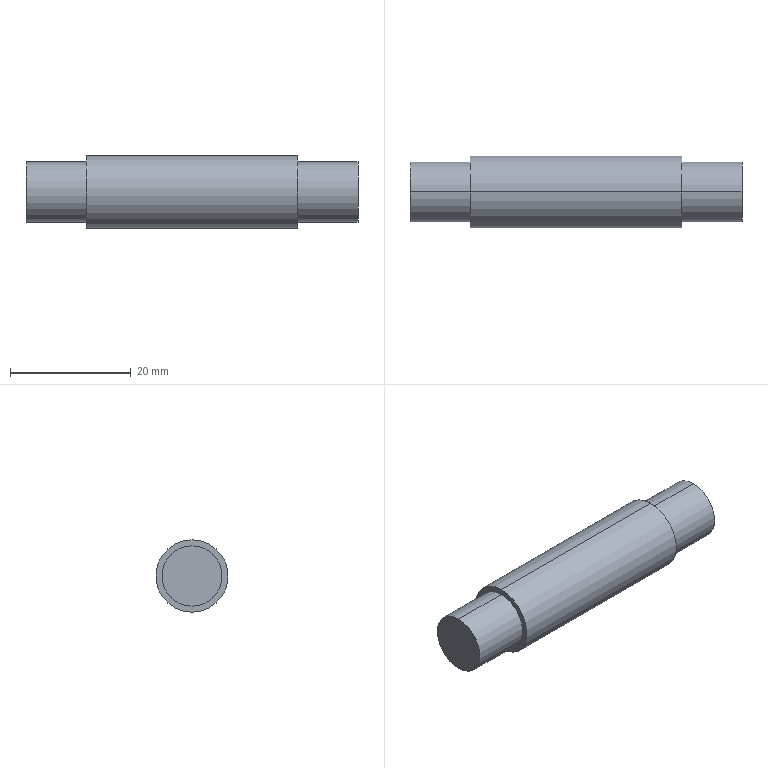Component | SolidWorks | CHEN123-AA-10-2 | 1 solid | 10 faces | box 55 x 12 x 12 mm | volume 5529 mm3 | cylinder 6 | plane 4 | commonest cylinder face diameters 10 x4 12 x2
build123d program:
from build123d import *

# Parameters (mm, degrees)
SKETCH1_R           = 6
BOSS_EXTRUDE1_DEPTH = 35
SKETCH2_R           = 5
BOSS_EXTRUDE2_DEPTH = 10
BOSS_EXTRUDE3_START = 10
SKETCH3_R           = 5
BOSS_EXTRUDE3_DEPTH = 10


with BuildPart() as part:
    # Sketch1 → Boss-Extrude1 (new body)
    with BuildSketch(Plane.XY):
        Circle(SKETCH1_R)
    extrude(amount=BOSS_EXTRUDE1_DEPTH)

    # Sketch2 → Boss-Extrude2 (add)
    with BuildSketch(Plane.XY.offset(35)):
        Circle(SKETCH2_R)
    extrude(amount=BOSS_EXTRUDE2_DEPTH)

    # Sketch3 → Boss-Extrude3 (add)
    with BuildSketch(Plane(origin=(0, 0, 0), x_dir=(-1, 0, 0), z_dir=(0, 0, -1)).offset(BOSS_EXTRUDE3_START)):
        with Locations(Location((0, 0, 0), (0, 0, 180))):
            Circle(SKETCH3_R)
    extrude(amount=-BOSS_EXTRUDE3_DEPTH)


solid = part.part

# Placed as in the assembly
solid = solid.moved(Location((-17, 4.001, -434), (0, 90, 0)))
STEP:
#1=COLOUR_RGB('',0.7922,0.8196,0.9333);
#2=FILL_AREA_STYLE_COLOUR('',#1);
#3=FILL_AREA_STYLE('',(#2));
#4=SURFACE_STYLE_FILL_AREA(#3);
#5=SURFACE_SIDE_STYLE('',(#4));
#6=SURFACE_STYLE_USAGE(.BOTH.,#5);
#7=PRESENTATION_STYLE_ASSIGNMENT((#6));
#8=CARTESIAN_POINT('',(-1.063,0.1575,-16.89));
#9=VERTEX_POINT('',#8);
#10=CARTESIAN_POINT('',(-1.063,0.1575,-17.283));
#11=VERTEX_POINT('',#10);
#12=CARTESIAN_POINT('',(-1.063,0.1575,-17.087));
#13=DIRECTION('',(-1.,0.,0.));
#14=DIRECTION('',(0.,0.,1.));
#15=AXIS2_PLACEMENT_3D('',#12,#13,#14);
#16=CIRCLE('',#15,0.1969);
#17=EDGE_CURVE('',#9,#11,#16,.T.);
#18=ORIENTED_EDGE('',*,*,#17,.F.);
#19=CARTESIAN_POINT('',(-0.6693,0.1575,-16.89));
#20=VERTEX_POINT('',#19);
#21=CARTESIAN_POINT('',(-1.063,0.1575,-16.89));
#22=DIRECTION('',(1.,0.,0.));
#23=VECTOR('',#22,39.37);
#24=LINE('',#21,#23);
#25=EDGE_CURVE('',#9,#20,#24,.T.);
#26=ORIENTED_EDGE('',*,*,#25,.T.);
#27=CARTESIAN_POINT('',(-0.6693,0.1575,-17.283));
#28=VERTEX_POINT('',#27);
#29=CARTESIAN_POINT('',(-0.6693,0.1575,-17.087));
#30=DIRECTION('',(-1.,0.,0.));
#31=DIRECTION('',(0.,0.,1.));
#32=AXIS2_PLACEMENT_3D('',#29,#30,#31);
#33=CIRCLE('',#32,0.1969);
#34=EDGE_CURVE('',#20,#28,#33,.T.);
#35=ORIENTED_EDGE('',*,*,#34,.T.);
#36=CARTESIAN_POINT('',(-1.063,0.1575,-17.283));
#37=DIRECTION('',(1.,0.,0.));
#38=VECTOR('',#37,39.37);
#39=LINE('',#36,#38);
#40=EDGE_CURVE('',#11,#28,#39,.T.);
#41=ORIENTED_EDGE('',*,*,#40,.F.);
#42=EDGE_LOOP('',(#18,#26,#35,#41));
#43=FACE_OUTER_BOUND('',#42,.T.);
#44=CARTESIAN_POINT('',(-1.063,0.1575,-17.087));
#45=DIRECTION('',(1.,0.,0.));
#46=DIRECTION('',(0.,0.,-1.));
#47=AXIS2_PLACEMENT_3D('',#44,#45,#46);
#48=CYLINDRICAL_SURFACE('',#47,0.1969);
#49=ADVANCED_FACE('',(#43),#48,.T.);
#50=CARTESIAN_POINT('',(1.102,0.1575,-17.283));
#51=VERTEX_POINT('',#50);
#52=CARTESIAN_POINT('',(1.102,0.1575,-16.89));
#53=VERTEX_POINT('',#52);
#54=CARTESIAN_POINT('',(1.102,0.1575,-17.087));
#55=DIRECTION('',(1.,0.,0.));
#56=DIRECTION('',(0.,0.,-1.));
#57=AXIS2_PLACEMENT_3D('',#54,#55,#56);
#58=CIRCLE('',#57,0.1969);
#59=EDGE_CURVE('',#51,#53,#58,.T.);
#60=ORIENTED_EDGE('',*,*,#59,.F.);
#61=CARTESIAN_POINT('',(0.7086,0.1575,-17.283));
#62=VERTEX_POINT('',#61);
#63=CARTESIAN_POINT('',(1.102,0.1575,-17.283));
#64=DIRECTION('',(-1.,0.,0.));
#65=VECTOR('',#64,39.37);
#66=LINE('',#63,#65);
#67=EDGE_CURVE('',#51,#62,#66,.T.);
#68=ORIENTED_EDGE('',*,*,#67,.T.);
#69=CARTESIAN_POINT('',(0.7086,0.1575,-16.89));
#70=VERTEX_POINT('',#69);
#71=CARTESIAN_POINT('',(0.7086,0.1575,-17.087));
#72=DIRECTION('',(1.,0.,0.));
#73=DIRECTION('',(0.,0.,-1.));
#74=AXIS2_PLACEMENT_3D('',#71,#72,#73);
#75=CIRCLE('',#74,0.1969);
#76=EDGE_CURVE('',#62,#70,#75,.T.);
#77=ORIENTED_EDGE('',*,*,#76,.T.);
#78=CARTESIAN_POINT('',(1.102,0.1575,-16.89));
#79=DIRECTION('',(-1.,0.,0.));
#80=VECTOR('',#79,39.37);
#81=LINE('',#78,#80);
#82=EDGE_CURVE('',#53,#70,#81,.T.);
#83=ORIENTED_EDGE('',*,*,#82,.F.);
#84=EDGE_LOOP('',(#60,#68,#77,#83));
#85=FACE_OUTER_BOUND('',#84,.T.);
#86=CARTESIAN_POINT('',(1.102,0.1575,-17.087));
#87=DIRECTION('',(-1.,0.,0.));
#88=DIRECTION('',(0.,0.,1.));
#89=AXIS2_PLACEMENT_3D('',#86,#87,#88);
#90=CYLINDRICAL_SURFACE('',#89,0.1969);
#91=ADVANCED_FACE('',(#85),#90,.T.);
#92=CARTESIAN_POINT('',(0.7086,0.1575,-17.323));
#93=VERTEX_POINT('',#92);
#94=CARTESIAN_POINT('',(0.7086,0.1575,-16.85));
#95=VERTEX_POINT('',#94);
#96=CARTESIAN_POINT('',(0.7086,0.1575,-17.087));
#97=DIRECTION('',(1.,0.,0.));
#98=DIRECTION('',(0.,0.,-1.));
#99=AXIS2_PLACEMENT_3D('',#96,#97,#98);
#100=CIRCLE('',#99,0.2362);
#101=EDGE_CURVE('',#93,#95,#100,.T.);
#102=ORIENTED_EDGE('',*,*,#101,.F.);
#103=CARTESIAN_POINT('',(-0.6693,0.1575,-17.323));
#104=VERTEX_POINT('',#103);
#105=CARTESIAN_POINT('',(0.7086,0.1575,-17.323));
#106=DIRECTION('',(-1.,0.,0.));
#107=VECTOR('',#106,39.37);
#108=LINE('',#105,#107);
#109=EDGE_CURVE('',#93,#104,#108,.T.);
#110=ORIENTED_EDGE('',*,*,#109,.T.);
#111=CARTESIAN_POINT('',(-0.6693,0.1575,-16.85));
#112=VERTEX_POINT('',#111);
#113=CARTESIAN_POINT('',(-0.6693,0.1575,-17.087));
#114=DIRECTION('',(1.,0.,0.));
#115=DIRECTION('',(0.,0.,-1.));
#116=AXIS2_PLACEMENT_3D('',#113,#114,#115);
#117=CIRCLE('',#116,0.2362);
#118=EDGE_CURVE('',#104,#112,#117,.T.);
#119=ORIENTED_EDGE('',*,*,#118,.T.);
#120=CARTESIAN_POINT('',(0.7086,0.1575,-16.85));
#121=DIRECTION('',(-1.,0.,0.));
#122=VECTOR('',#121,39.37);
#123=LINE('',#120,#122);
#124=EDGE_CURVE('',#95,#112,#123,.T.);
#125=ORIENTED_EDGE('',*,*,#124,.F.);
#126=EDGE_LOOP('',(#102,#110,#119,#125));
#127=FACE_OUTER_BOUND('',#126,.T.);
#128=CARTESIAN_POINT('',(0.7086,0.1575,-17.087));
#129=DIRECTION('',(-1.,0.,0.));
#130=DIRECTION('',(0.,0.,1.));
#131=AXIS2_PLACEMENT_3D('',#128,#129,#130);
#132=CYLINDRICAL_SURFACE('',#131,0.2362);
#133=ADVANCED_FACE('',(#127),#132,.T.);
#134=ORIENTED_EDGE('',*,*,#109,.F.);
#135=CARTESIAN_POINT('',(0.7086,0.1575,-17.087));
#136=DIRECTION('',(1.,0.,0.));
#137=DIRECTION('',(0.,0.,-1.));
#138=AXIS2_PLACEMENT_3D('',#135,#136,#137);
#139=CIRCLE('',#138,0.2362);
#140=EDGE_CURVE('',#95,#93,#139,.T.);
#141=ORIENTED_EDGE('',*,*,#140,.F.);
#142=ORIENTED_EDGE('',*,*,#124,.T.);
#143=CARTESIAN_POINT('',(-0.6693,0.1575,-17.087));
#144=DIRECTION('',(1.,0.,0.));
#145=DIRECTION('',(0.,0.,-1.));
#146=AXIS2_PLACEMENT_3D('',#143,#144,#145);
#147=CIRCLE('',#146,0.2362);
#148=EDGE_CURVE('',#112,#104,#147,.T.);
#149=ORIENTED_EDGE('',*,*,#148,.T.);
#150=EDGE_LOOP('',(#134,#141,#142,#149));
#151=FACE_OUTER_BOUND('',#150,.T.);
#152=CARTESIAN_POINT('',(0.7086,0.1575,-17.087));
#153=DIRECTION('',(-1.,0.,0.));
#154=DIRECTION('',(0.,0.,1.));
#155=AXIS2_PLACEMENT_3D('',#152,#153,#154);
#156=CYLINDRICAL_SURFACE('',#155,0.2362);
#157=ADVANCED_FACE('',(#151),#156,.T.);
#158=CARTESIAN_POINT('',(0.7086,0.1575,-17.087));
#159=DIRECTION('',(1.,0.,0.));
#160=DIRECTION('',(0.,0.,-1.));
#161=AXIS2_PLACEMENT_3D('',#158,#159,#160);
#162=CIRCLE('',#161,0.1969);
#163=EDGE_CURVE('',#70,#62,#162,.T.);
#164=ORIENTED_EDGE('',*,*,#163,.F.);
#165=ORIENTED_EDGE('',*,*,#76,.F.);
#166=EDGE_LOOP('',(#164,#165));
#167=FACE_BOUND('',#166,.T.);
#168=ORIENTED_EDGE('',*,*,#140,.T.);
#169=ORIENTED_EDGE('',*,*,#101,.T.);
#170=EDGE_LOOP('',(#168,#169));
#171=FACE_OUTER_BOUND('',#170,.T.);
#172=CARTESIAN_POINT('',(0.7086,0.1575,-17.087));
#173=DIRECTION('',(1.,0.,0.));
#174=DIRECTION('',(0.,0.,-1.));
#175=AXIS2_PLACEMENT_3D('',#172,#173,#174);
#176=PLANE('',#175);
#177=ADVANCED_FACE('',(#167,#171),#176,.T.);
#178=CARTESIAN_POINT('',(-0.6693,0.1575,-17.087));
#179=DIRECTION('',(-1.,0.,0.));
#180=DIRECTION('',(0.,0.,1.));
#181=AXIS2_PLACEMENT_3D('',#178,#179,#180);
#182=CIRCLE('',#181,0.1969);
#183=EDGE_CURVE('',#28,#20,#182,.T.);
#184=ORIENTED_EDGE('',*,*,#183,.F.);
#185=ORIENTED_EDGE('',*,*,#34,.F.);
#186=EDGE_LOOP('',(#184,#185));
#187=FACE_BOUND('',#186,.T.);
#188=ORIENTED_EDGE('',*,*,#148,.F.);
#189=ORIENTED_EDGE('',*,*,#118,.F.);
#190=EDGE_LOOP('',(#188,#189));
#191=FACE_OUTER_BOUND('',#190,.T.);
#192=CARTESIAN_POINT('',(-0.6693,0.1575,-17.087));
#193=DIRECTION('',(1.,0.,0.));
#194=DIRECTION('',(0.,0.,-1.));
#195=AXIS2_PLACEMENT_3D('',#192,#193,#194);
#196=PLANE('',#195);
#197=ADVANCED_FACE('',(#187,#191),#196,.F.);
#198=ORIENTED_EDGE('',*,*,#67,.F.);
#199=CARTESIAN_POINT('',(1.102,0.1575,-17.087));
#200=DIRECTION('',(1.,0.,0.));
#201=DIRECTION('',(0.,0.,-1.));
#202=AXIS2_PLACEMENT_3D('',#199,#200,#201);
#203=CIRCLE('',#202,0.1969);
#204=EDGE_CURVE('',#53,#51,#203,.T.);
#205=ORIENTED_EDGE('',*,*,#204,.F.);
#206=ORIENTED_EDGE('',*,*,#82,.T.);
#207=ORIENTED_EDGE('',*,*,#163,.T.);
#208=EDGE_LOOP('',(#198,#205,#206,#207));
#209=FACE_OUTER_BOUND('',#208,.T.);
#210=CARTESIAN_POINT('',(1.102,0.1575,-17.087));
#211=DIRECTION('',(-1.,0.,0.));
#212=DIRECTION('',(0.,0.,1.));
#213=AXIS2_PLACEMENT_3D('',#210,#211,#212);
#214=CYLINDRICAL_SURFACE('',#213,0.1969);
#215=ADVANCED_FACE('',(#209),#214,.T.);
#216=ORIENTED_EDGE('',*,*,#204,.T.);
#217=ORIENTED_EDGE('',*,*,#59,.T.);
#218=EDGE_LOOP('',(#216,#217));
#219=FACE_OUTER_BOUND('',#218,.T.);
#220=CARTESIAN_POINT('',(1.102,0.1575,-17.087));
#221=DIRECTION('',(1.,0.,0.));
#222=DIRECTION('',(0.,0.,-1.));
#223=AXIS2_PLACEMENT_3D('',#220,#221,#222);
#224=PLANE('',#223);
#225=ADVANCED_FACE('',(#219),#224,.T.);
#226=ORIENTED_EDGE('',*,*,#25,.F.);
#227=CARTESIAN_POINT('',(-1.063,0.1575,-17.087));
#228=DIRECTION('',(-1.,0.,0.));
#229=DIRECTION('',(0.,0.,1.));
#230=AXIS2_PLACEMENT_3D('',#227,#228,#229);
#231=CIRCLE('',#230,0.1969);
#232=EDGE_CURVE('',#11,#9,#231,.T.);
#233=ORIENTED_EDGE('',*,*,#232,.F.);
#234=ORIENTED_EDGE('',*,*,#40,.T.);
#235=ORIENTED_EDGE('',*,*,#183,.T.);
#236=EDGE_LOOP('',(#226,#233,#234,#235));
#237=FACE_OUTER_BOUND('',#236,.T.);
#238=CARTESIAN_POINT('',(-1.063,0.1575,-17.087));
#239=DIRECTION('',(1.,0.,0.));
#240=DIRECTION('',(0.,0.,-1.));
#241=AXIS2_PLACEMENT_3D('',#238,#239,#240);
#242=CYLINDRICAL_SURFACE('',#241,0.1969);
#243=ADVANCED_FACE('',(#237),#242,.T.);
#244=ORIENTED_EDGE('',*,*,#232,.T.);
#245=ORIENTED_EDGE('',*,*,#17,.T.);
#246=EDGE_LOOP('',(#244,#245));
#247=FACE_OUTER_BOUND('',#246,.T.);
#248=CARTESIAN_POINT('',(-1.063,0.1575,-17.087));
#249=DIRECTION('',(-1.,0.,0.));
#250=DIRECTION('',(0.,0.,1.));
#251=AXIS2_PLACEMENT_3D('',#248,#249,#250);
#252=PLANE('',#251);
#253=ADVANCED_FACE('',(#247),#252,.T.);
#254=CLOSED_SHELL('',(#49,#91,#133,#157,#177,#197,#215,#225,#243,#253));
#255=MANIFOLD_SOLID_BREP('',#254);
#256=STYLED_ITEM('',(#7),#255);
#257=(LENGTH_UNIT()NAMED_UNIT(*)SI_UNIT($,.METRE.));
#258=LENGTH_MEASURE_WITH_UNIT(LENGTH_MEASURE(0.0254),#257);
#259=DIMENSIONAL_EXPONENTS(1.,0.,0.,0.,0.,0.,0.);
#260=(CONVERSION_BASED_UNIT('',#258)LENGTH_UNIT()NAMED_UNIT(#259));
#261=UNCERTAINTY_MEASURE_WITH_UNIT(LENGTH_MEASURE(0.00001),#260,'','');
#262=(NAMED_UNIT(*)PLANE_ANGLE_UNIT()SI_UNIT($,.RADIAN.));
#263=(NAMED_UNIT(*)SI_UNIT($,.STERADIAN.)SOLID_ANGLE_UNIT());
#264=(GEOMETRIC_REPRESENTATION_CONTEXT(3)GLOBAL_UNCERTAINTY_ASSIGNED_CONTEXT((#261))GLOBAL_UNIT_ASSIGNED_CONTEXT((#260,#262,#263))REPRESENTATION_CONTEXT('',''));
#265=MECHANICAL_DESIGN_GEOMETRIC_PRESENTATION_REPRESENTATION('',(#256),#264);
#266=PRESENTATION_LAYER_ASSIGNMENT('','',(#256));
#267=CARTESIAN_POINT('',(0.,0.,0.));
#268=DIRECTION('',(0.,0.,1.));
#269=DIRECTION('',(1.,0.,0.));
#270=AXIS2_PLACEMENT_3D('',#267,#268,#269);
#271=(LENGTH_UNIT()NAMED_UNIT(*)SI_UNIT($,.METRE.));
#272=LENGTH_MEASURE_WITH_UNIT(LENGTH_MEASURE(0.0254),#271);
#273=DIMENSIONAL_EXPONENTS(1.,0.,0.,0.,0.,0.,0.);
#274=(CONVERSION_BASED_UNIT('',#272)LENGTH_UNIT()NAMED_UNIT(#273));
#275=UNCERTAINTY_MEASURE_WITH_UNIT(LENGTH_MEASURE(0.00001),#274,'','');
#276=(NAMED_UNIT(*)PLANE_ANGLE_UNIT()SI_UNIT($,.RADIAN.));
#277=(NAMED_UNIT(*)SI_UNIT($,.STERADIAN.)SOLID_ANGLE_UNIT());
#278=(GEOMETRIC_REPRESENTATION_CONTEXT(3)GLOBAL_UNCERTAINTY_ASSIGNED_CONTEXT((#275))GLOBAL_UNIT_ASSIGNED_CONTEXT((#274,#276,#277))REPRESENTATION_CONTEXT('',''));
#279=ADVANCED_BREP_SHAPE_REPRESENTATION('',(#255,#270),#278);